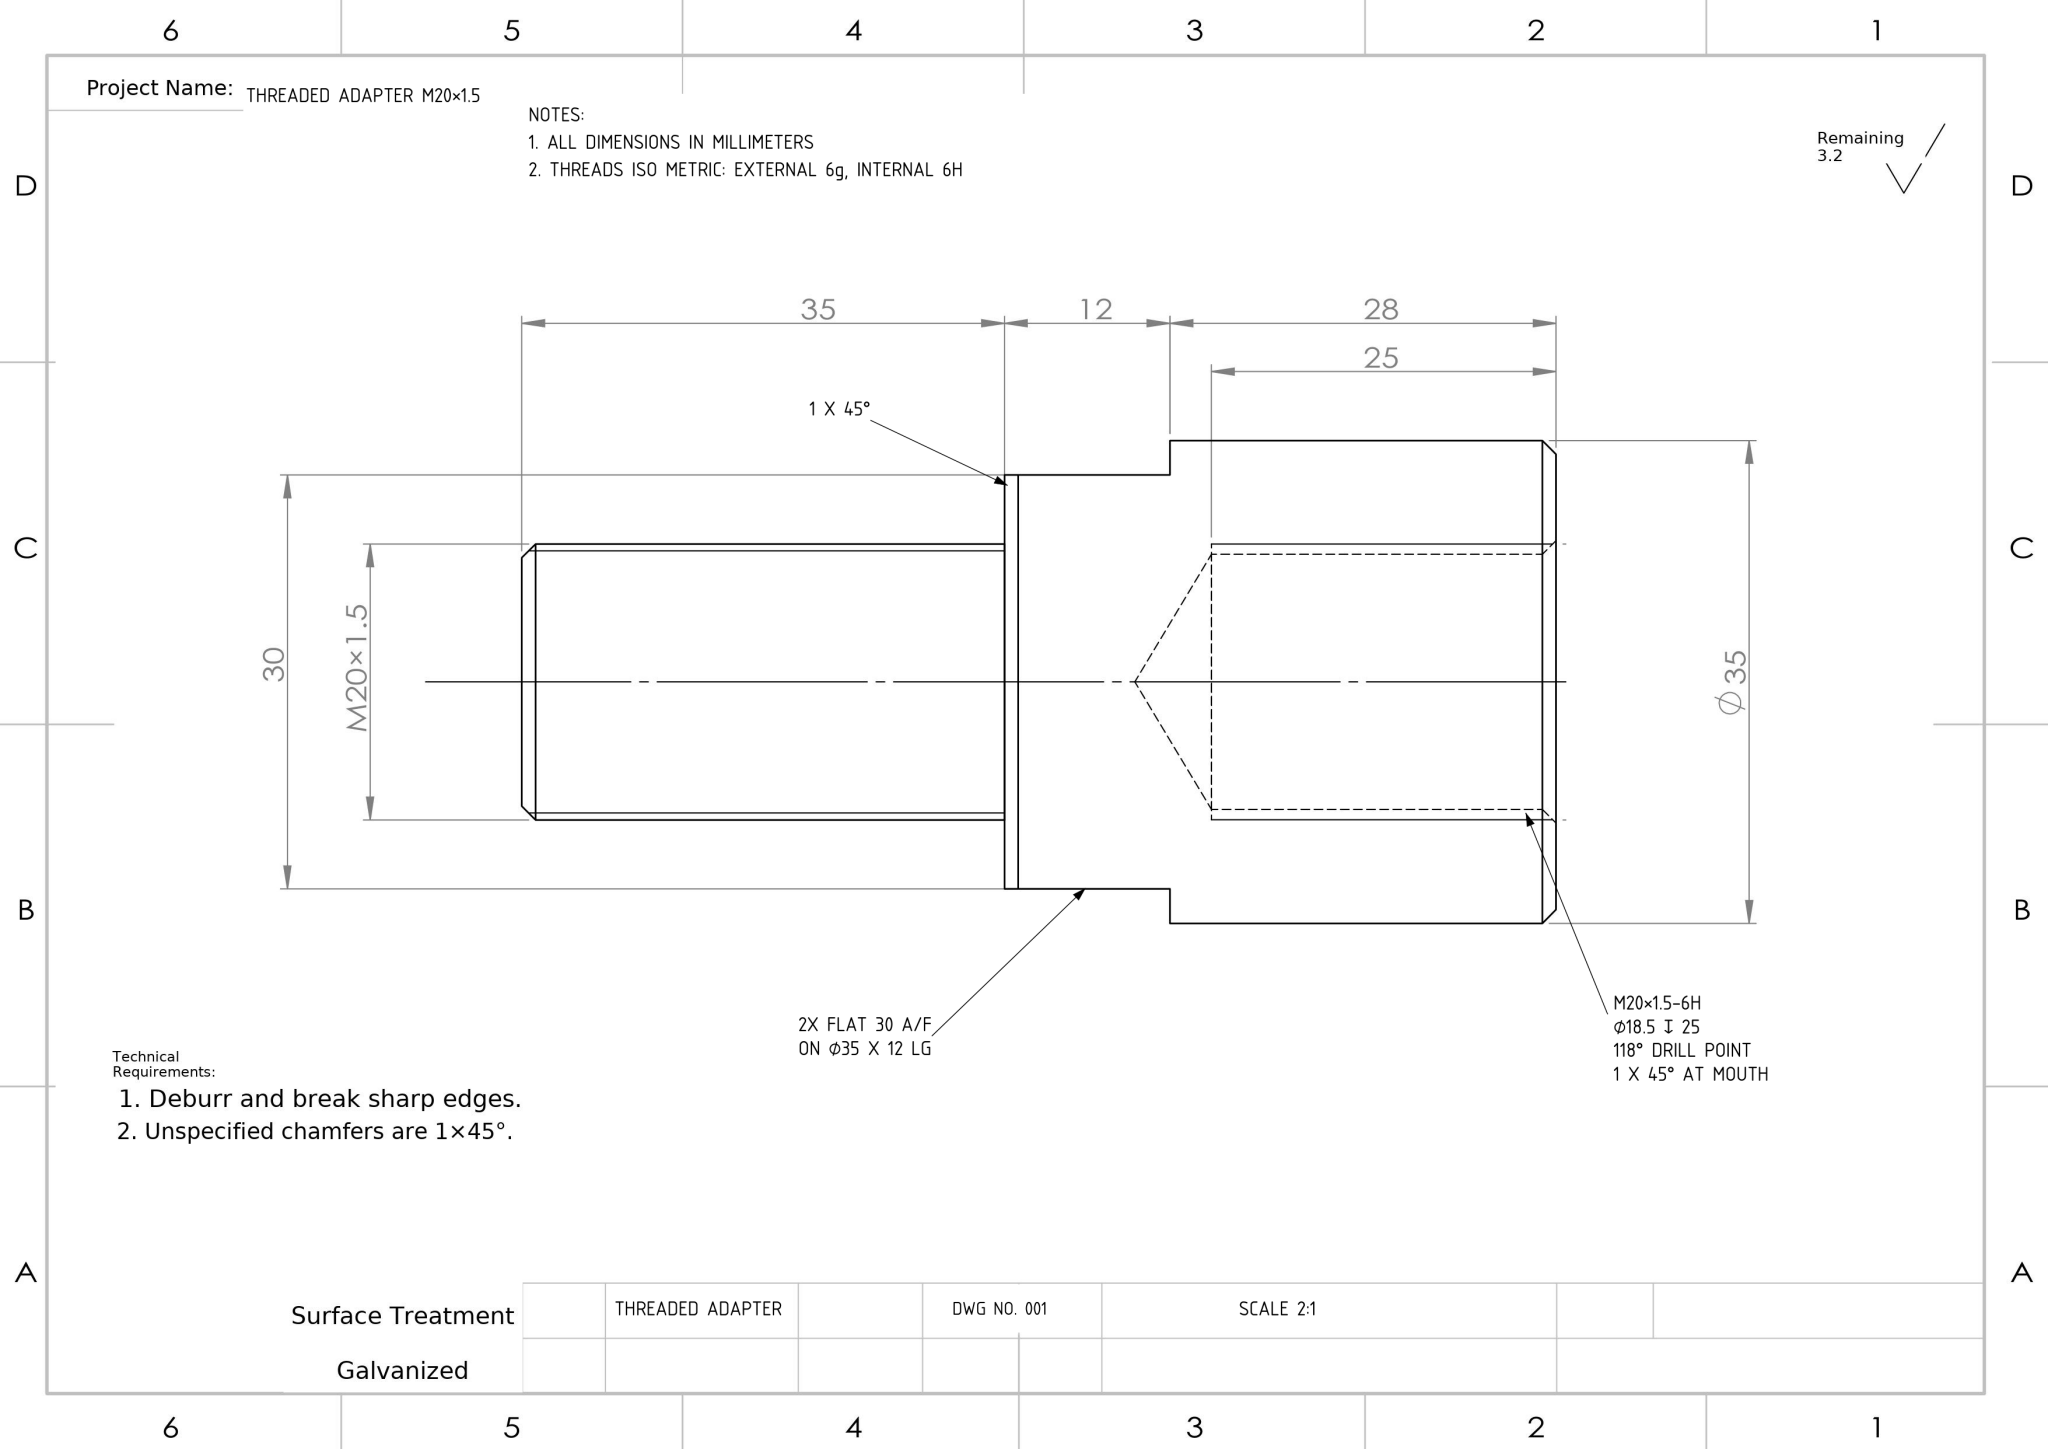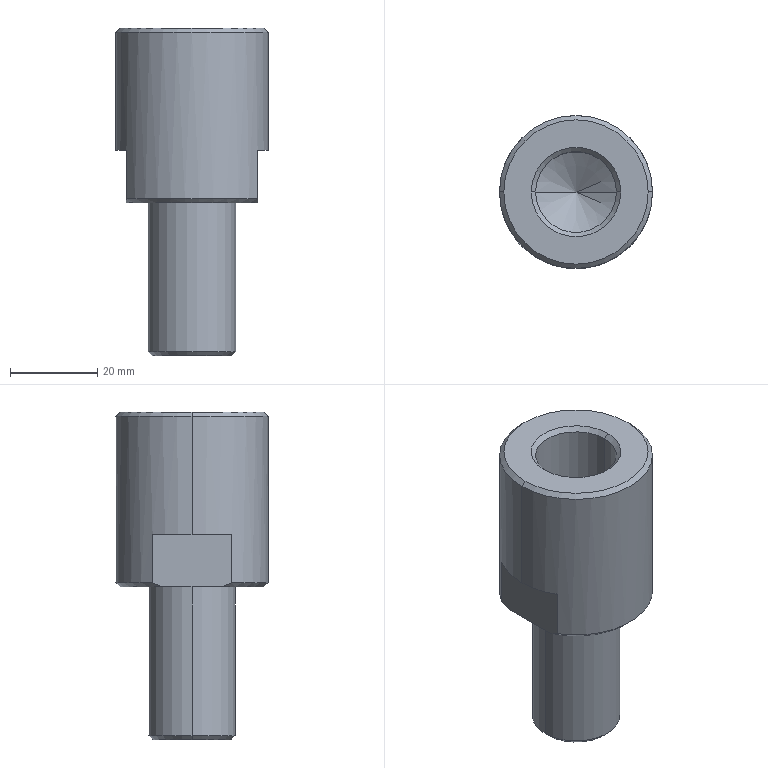Part | NX | mm | 1 solid | 23 faces | box 35 x 35 x 75 mm | volume 41379 mm3 | cone 10 | plane 7 | cylinder 6 | commonest cylinder face diameters 18.5 x2 35 x2 20 x2
STEP:
#1=COLOUR_RGB('',0.7529,0.7529,0.7529);
#2=FILL_AREA_STYLE_COLOUR('',#1);
#3=FILL_AREA_STYLE('',(#2));
#4=SURFACE_STYLE_FILL_AREA(#3);
#5=SURFACE_SIDE_STYLE('',(#4));
#6=SURFACE_STYLE_USAGE(.BOTH.,#5);
#7=PRESENTATION_STYLE_ASSIGNMENT((#6));
#8=CARTESIAN_POINT('',(-9.25,0.,50.));
#9=VERTEX_POINT('',#8);
#10=CARTESIAN_POINT('',(-9.25,0.,74.));
#11=VERTEX_POINT('',#10);
#12=CARTESIAN_POINT('',(-9.25,0.,75.));
#13=DIRECTION('',(0.,0.,1.));
#14=VECTOR('',#13,1000.);
#15=LINE('',#12,#14);
#16=EDGE_CURVE('',#9,#11,#15,.T.);
#17=ORIENTED_EDGE('',*,*,#16,.F.);
#18=CARTESIAN_POINT('',(9.25,0.,50.));
#19=VERTEX_POINT('',#18);
#20=CARTESIAN_POINT('',(0.,0.,50.));
#21=DIRECTION('',(0.,0.,1.));
#22=DIRECTION('',(1.,0.,0.));
#23=AXIS2_PLACEMENT_3D('',#20,#21,#22);
#24=CIRCLE('',#23,9.25);
#25=EDGE_CURVE('',#19,#9,#24,.T.);
#26=ORIENTED_EDGE('',*,*,#25,.F.);
#27=CARTESIAN_POINT('',(9.25,0.,74.));
#28=VERTEX_POINT('',#27);
#29=CARTESIAN_POINT('',(9.25,0.,75.));
#30=DIRECTION('',(0.,0.,1.));
#31=VECTOR('',#30,1000.);
#32=LINE('',#29,#31);
#33=EDGE_CURVE('',#19,#28,#32,.T.);
#34=ORIENTED_EDGE('',*,*,#33,.T.);
#35=CARTESIAN_POINT('',(0.,0.,74.));
#36=DIRECTION('',(0.,0.,1.));
#37=DIRECTION('',(1.,0.,0.));
#38=AXIS2_PLACEMENT_3D('',#35,#36,#37);
#39=CIRCLE('',#38,9.25);
#40=EDGE_CURVE('',#28,#11,#39,.T.);
#41=ORIENTED_EDGE('',*,*,#40,.T.);
#42=EDGE_LOOP('',(#17,#26,#34,#41));
#43=FACE_OUTER_BOUND('',#42,.T.);
#44=CARTESIAN_POINT('',(0.,0.,75.));
#45=DIRECTION('',(0.,0.,1.));
#46=DIRECTION('',(1.,0.,0.));
#47=AXIS2_PLACEMENT_3D('',#44,#45,#46);
#48=CYLINDRICAL_SURFACE('',#47,9.25);
#49=ADVANCED_FACE('',(#43),#48,.F.);
#50=STYLED_ITEM('',(#7),#49);
#51=(LENGTH_UNIT()NAMED_UNIT(*)SI_UNIT(.MILLI.,.METRE.));
#52=UNCERTAINTY_MEASURE_WITH_UNIT(LENGTH_MEASURE(0.00001),#51,'','');
#53=(NAMED_UNIT(*)PLANE_ANGLE_UNIT()SI_UNIT($,.RADIAN.));
#54=(NAMED_UNIT(*)SI_UNIT($,.STERADIAN.)SOLID_ANGLE_UNIT());
#55=(GEOMETRIC_REPRESENTATION_CONTEXT(3)GLOBAL_UNCERTAINTY_ASSIGNED_CONTEXT((#52))GLOBAL_UNIT_ASSIGNED_CONTEXT((#51,#53,#54))REPRESENTATION_CONTEXT('',''));
#56=MECHANICAL_DESIGN_GEOMETRIC_PRESENTATION_REPRESENTATION('',(#50),#55);
#57=PRESENTATION_LAYER_ASSIGNMENT('','',(#50));
#58=COLOUR_RGB('',0.7529,0.7529,0.7529);
#59=FILL_AREA_STYLE_COLOUR('',#58);
#60=FILL_AREA_STYLE('',(#59));
#61=SURFACE_STYLE_FILL_AREA(#60);
#62=SURFACE_SIDE_STYLE('',(#61));
#63=SURFACE_STYLE_USAGE(.BOTH.,#62);
#64=PRESENTATION_STYLE_ASSIGNMENT((#63));
#65=CARTESIAN_POINT('',(0.,0.,50.));
#66=DIRECTION('',(0.,0.,1.));
#67=DIRECTION('',(1.,0.,0.));
#68=AXIS2_PLACEMENT_3D('',#65,#66,#67);
#69=CIRCLE('',#68,9.25);
#70=EDGE_CURVE('',#9,#19,#69,.T.);
#71=ORIENTED_EDGE('',*,*,#70,.F.);
#72=ORIENTED_EDGE('',*,*,#16,.T.);
#73=CARTESIAN_POINT('',(0.,0.,74.));
#74=DIRECTION('',(0.,0.,1.));
#75=DIRECTION('',(1.,0.,0.));
#76=AXIS2_PLACEMENT_3D('',#73,#74,#75);
#77=CIRCLE('',#76,9.25);
#78=EDGE_CURVE('',#11,#28,#77,.T.);
#79=ORIENTED_EDGE('',*,*,#78,.T.);
#80=ORIENTED_EDGE('',*,*,#33,.F.);
#81=EDGE_LOOP('',(#71,#72,#79,#80));
#82=FACE_OUTER_BOUND('',#81,.T.);
#83=CARTESIAN_POINT('',(0.,0.,75.));
#84=DIRECTION('',(0.,0.,1.));
#85=DIRECTION('',(1.,0.,0.));
#86=AXIS2_PLACEMENT_3D('',#83,#84,#85);
#87=CYLINDRICAL_SURFACE('',#86,9.25);
#88=ADVANCED_FACE('',(#82),#87,.F.);
#89=STYLED_ITEM('',(#64),#88);
#90=PRESENTATION_LAYER_ASSIGNMENT('','',(#89));
#91=COLOUR_RGB('',0.7529,0.7529,0.7529);
#92=FILL_AREA_STYLE_COLOUR('',#91);
#93=FILL_AREA_STYLE('',(#92));
#94=SURFACE_STYLE_FILL_AREA(#93);
#95=SURFACE_SIDE_STYLE('',(#94));
#96=SURFACE_STYLE_USAGE(.BOTH.,#95);
#97=PRESENTATION_STYLE_ASSIGNMENT((#96));
#98=ORIENTED_EDGE('',*,*,#78,.F.);
#99=CARTESIAN_POINT('',(-10.25,0.,75.));
#100=VERTEX_POINT('',#99);
#101=CARTESIAN_POINT('',(-9.25,0.,74.));
#102=DIRECTION('',(-0.7071,0.,0.7071));
#103=VECTOR('',#102,1000.);
#104=LINE('',#101,#103);
#105=EDGE_CURVE('',#11,#100,#104,.T.);
#106=ORIENTED_EDGE('',*,*,#105,.T.);
#107=CARTESIAN_POINT('',(10.25,0.,75.));
#108=VERTEX_POINT('',#107);
#109=CARTESIAN_POINT('',(0.,0.,75.));
#110=DIRECTION('',(0.,0.,-1.));
#111=DIRECTION('',(1.,0.,0.));
#112=AXIS2_PLACEMENT_3D('',#109,#110,#111);
#113=CIRCLE('',#112,10.25);
#114=EDGE_CURVE('',#108,#100,#113,.T.);
#115=ORIENTED_EDGE('',*,*,#114,.F.);
#116=CARTESIAN_POINT('',(9.25,0.,74.));
#117=DIRECTION('',(0.7071,0.,0.7071));
#118=VECTOR('',#117,1000.);
#119=LINE('',#116,#118);
#120=EDGE_CURVE('',#28,#108,#119,.T.);
#121=ORIENTED_EDGE('',*,*,#120,.F.);
#122=EDGE_LOOP('',(#98,#106,#115,#121));
#123=FACE_OUTER_BOUND('',#122,.T.);
#124=CARTESIAN_POINT('',(0.,0.,74.));
#125=DIRECTION('',(0.,0.,1.));
#126=DIRECTION('',(1.,0.,0.));
#127=AXIS2_PLACEMENT_3D('',#124,#125,#126);
#128=CONICAL_SURFACE('',#127,9.25,0.7854);
#129=ADVANCED_FACE('',(#123),#128,.F.);
#130=CARTESIAN_POINT('',(-0.,0.,44.442));
#131=VERTEX_POINT('',#130);
#132=CARTESIAN_POINT('',(9.25,0.,50.));
#133=DIRECTION('',(0.8572,0.,0.515));
#134=VECTOR('',#133,1000.);
#135=LINE('',#132,#134);
#136=EDGE_CURVE('',#131,#19,#135,.T.);
#137=ORIENTED_EDGE('',*,*,#136,.F.);
#138=CARTESIAN_POINT('',(-9.25,0.,50.));
#139=DIRECTION('',(-0.8572,0.,0.515));
#140=VECTOR('',#139,1000.);
#141=LINE('',#138,#140);
#142=EDGE_CURVE('',#131,#9,#141,.T.);
#143=ORIENTED_EDGE('',*,*,#142,.T.);
#144=ORIENTED_EDGE('',*,*,#70,.T.);
#145=EDGE_LOOP('',(#137,#143,#144));
#146=FACE_OUTER_BOUND('',#145,.T.);
#147=CARTESIAN_POINT('',(0.,0.,50.));
#148=DIRECTION('',(0.,0.,1.));
#149=DIRECTION('',(1.,0.,0.));
#150=AXIS2_PLACEMENT_3D('',#147,#148,#149);
#151=CONICAL_SURFACE('',#150,9.25,1.03);
#152=ADVANCED_FACE('',(#146),#151,.F.);
#153=CARTESIAN_POINT('',(-9.,0.,0.));
#154=VERTEX_POINT('',#153);
#155=CARTESIAN_POINT('',(9.,0.,0.));
#156=VERTEX_POINT('',#155);
#157=CARTESIAN_POINT('',(0.,0.,0.));
#158=DIRECTION('',(0.,0.,-1.));
#159=DIRECTION('',(1.,0.,0.));
#160=AXIS2_PLACEMENT_3D('',#157,#158,#159);
#161=CIRCLE('',#160,9.);
#162=EDGE_CURVE('',#154,#156,#161,.T.);
#163=ORIENTED_EDGE('',*,*,#162,.F.);
#164=CARTESIAN_POINT('',(-10.,0.,1.));
#165=VERTEX_POINT('',#164);
#166=CARTESIAN_POINT('',(-10.,0.,1.));
#167=DIRECTION('',(-0.7071,0.,0.7071));
#168=VECTOR('',#167,1000.);
#169=LINE('',#166,#168);
#170=EDGE_CURVE('',#154,#165,#169,.T.);
#171=ORIENTED_EDGE('',*,*,#170,.T.);
#172=CARTESIAN_POINT('',(10.,0.,1.));
#173=VERTEX_POINT('',#172);
#174=CARTESIAN_POINT('',(0.,0.,1.));
#175=DIRECTION('',(0.,0.,1.));
#176=DIRECTION('',(1.,0.,0.));
#177=AXIS2_PLACEMENT_3D('',#174,#175,#176);
#178=CIRCLE('',#177,10.);
#179=EDGE_CURVE('',#173,#165,#178,.T.);
#180=ORIENTED_EDGE('',*,*,#179,.F.);
#181=CARTESIAN_POINT('',(10.,0.,1.));
#182=DIRECTION('',(0.7071,0.,0.7071));
#183=VECTOR('',#182,1000.);
#184=LINE('',#181,#183);
#185=EDGE_CURVE('',#156,#173,#184,.T.);
#186=ORIENTED_EDGE('',*,*,#185,.F.);
#187=EDGE_LOOP('',(#163,#171,#180,#186));
#188=FACE_OUTER_BOUND('',#187,.T.);
#189=CARTESIAN_POINT('',(0.,0.,1.));
#190=DIRECTION('',(0.,0.,1.));
#191=DIRECTION('',(1.,0.,0.));
#192=AXIS2_PLACEMENT_3D('',#189,#190,#191);
#193=CONICAL_SURFACE('',#192,10.,0.7854);
#194=ADVANCED_FACE('',(#188),#193,.T.);
#195=CARTESIAN_POINT('',(16.5,0.,75.));
#196=VERTEX_POINT('',#195);
#197=CARTESIAN_POINT('',(-16.5,0.,75.));
#198=VERTEX_POINT('',#197);
#199=CARTESIAN_POINT('',(0.,0.,75.));
#200=DIRECTION('',(0.,0.,1.));
#201=DIRECTION('',(1.,0.,0.));
#202=AXIS2_PLACEMENT_3D('',#199,#200,#201);
#203=CIRCLE('',#202,16.5);
#204=EDGE_CURVE('',#196,#198,#203,.T.);
#205=ORIENTED_EDGE('',*,*,#204,.F.);
#206=CARTESIAN_POINT('',(17.5,0.,74.));
#207=VERTEX_POINT('',#206);
#208=CARTESIAN_POINT('',(16.5,0.,75.));
#209=DIRECTION('',(0.7071,0.,-0.7071));
#210=VECTOR('',#209,1000.);
#211=LINE('',#208,#210);
#212=EDGE_CURVE('',#196,#207,#211,.T.);
#213=ORIENTED_EDGE('',*,*,#212,.T.);
#214=CARTESIAN_POINT('',(-17.5,0.,74.));
#215=VERTEX_POINT('',#214);
#216=CARTESIAN_POINT('',(0.,0.,74.));
#217=DIRECTION('',(0.,0.,-1.));
#218=DIRECTION('',(1.,0.,0.));
#219=AXIS2_PLACEMENT_3D('',#216,#217,#218);
#220=CIRCLE('',#219,17.5);
#221=EDGE_CURVE('',#215,#207,#220,.T.);
#222=ORIENTED_EDGE('',*,*,#221,.F.);
#223=CARTESIAN_POINT('',(-16.5,0.,75.));
#224=DIRECTION('',(-0.7071,0.,-0.7071));
#225=VECTOR('',#224,1000.);
#226=LINE('',#223,#225);
#227=EDGE_CURVE('',#198,#215,#226,.T.);
#228=ORIENTED_EDGE('',*,*,#227,.F.);
#229=EDGE_LOOP('',(#205,#213,#222,#228));
#230=FACE_OUTER_BOUND('',#229,.T.);
#231=CARTESIAN_POINT('',(0.,0.,75.));
#232=DIRECTION('',(0.,0.,-1.));
#233=DIRECTION('',(-1.,0.,0.));
#234=AXIS2_PLACEMENT_3D('',#231,#232,#233);
#235=CONICAL_SURFACE('',#234,16.5,0.7854);
#236=ADVANCED_FACE('',(#230),#235,.T.);
#237=ORIENTED_EDGE('',*,*,#221,.T.);
#238=CARTESIAN_POINT('',(17.5,0.,47.));
#239=VERTEX_POINT('',#238);
#240=CARTESIAN_POINT('',(17.5,0.,75.));
#241=DIRECTION('',(0.,0.,-1.));
#242=VECTOR('',#241,1000.);
#243=LINE('',#240,#242);
#244=EDGE_CURVE('',#207,#239,#243,.T.);
#245=ORIENTED_EDGE('',*,*,#244,.T.);
#246=CARTESIAN_POINT('',(15.,9.014,47.));
#247=VERTEX_POINT('',#246);
#248=CARTESIAN_POINT('',(0.,0.,47.));
#249=DIRECTION('',(0.,0.,1.));
#250=DIRECTION('',(1.,0.,0.));
#251=AXIS2_PLACEMENT_3D('',#248,#249,#250);
#252=CIRCLE('',#251,17.5);
#253=EDGE_CURVE('',#239,#247,#252,.T.);
#254=ORIENTED_EDGE('',*,*,#253,.T.);
#255=CARTESIAN_POINT('',(15.,9.014,36.));
#256=VERTEX_POINT('',#255);
#257=CARTESIAN_POINT('',(15.,9.014,75.));
#258=DIRECTION('',(0.,0.,-1.));
#259=VECTOR('',#258,1000.);
#260=LINE('',#257,#259);
#261=EDGE_CURVE('',#247,#256,#260,.T.);
#262=ORIENTED_EDGE('',*,*,#261,.T.);
#263=CARTESIAN_POINT('',(-15.,9.014,36.));
#264=VERTEX_POINT('',#263);
#265=CARTESIAN_POINT('',(0.,0.,36.));
#266=DIRECTION('',(0.,0.,1.));
#267=DIRECTION('',(1.,0.,0.));
#268=AXIS2_PLACEMENT_3D('',#265,#266,#267);
#269=CIRCLE('',#268,17.5);
#270=EDGE_CURVE('',#256,#264,#269,.T.);
#271=ORIENTED_EDGE('',*,*,#270,.T.);
#272=CARTESIAN_POINT('',(-15.,9.014,47.));
#273=VERTEX_POINT('',#272);
#274=CARTESIAN_POINT('',(-15.,9.014,75.));
#275=DIRECTION('',(0.,0.,1.));
#276=VECTOR('',#275,1000.);
#277=LINE('',#274,#276);
#278=EDGE_CURVE('',#264,#273,#277,.T.);
#279=ORIENTED_EDGE('',*,*,#278,.T.);
#280=CARTESIAN_POINT('',(-17.5,0.,47.));
#281=VERTEX_POINT('',#280);
#282=CARTESIAN_POINT('',(0.,0.,47.));
#283=DIRECTION('',(0.,0.,1.));
#284=DIRECTION('',(1.,0.,0.));
#285=AXIS2_PLACEMENT_3D('',#282,#283,#284);
#286=CIRCLE('',#285,17.5);
#287=EDGE_CURVE('',#273,#281,#286,.T.);
#288=ORIENTED_EDGE('',*,*,#287,.T.);
#289=CARTESIAN_POINT('',(-17.5,0.,75.));
#290=DIRECTION('',(0.,0.,-1.));
#291=VECTOR('',#290,1000.);
#292=LINE('',#289,#291);
#293=EDGE_CURVE('',#215,#281,#292,.T.);
#294=ORIENTED_EDGE('',*,*,#293,.F.);
#295=EDGE_LOOP('',(#237,#245,#254,#262,#271,#279,#288,#294));
#296=FACE_OUTER_BOUND('',#295,.T.);
#297=CARTESIAN_POINT('',(0.,0.,75.));
#298=DIRECTION('',(0.,0.,-1.));
#299=DIRECTION('',(-1.,0.,0.));
#300=AXIS2_PLACEMENT_3D('',#297,#298,#299);
#301=CYLINDRICAL_SURFACE('',#300,17.5);
#302=ADVANCED_FACE('',(#296),#301,.T.);
#303=CARTESIAN_POINT('',(10.,0.,35.));
#304=VERTEX_POINT('',#303);
#305=CARTESIAN_POINT('',(-10.,0.,35.));
#306=VERTEX_POINT('',#305);
#307=CARTESIAN_POINT('',(0.,0.,35.));
#308=DIRECTION('',(0.,0.,1.));
#309=DIRECTION('',(1.,0.,0.));
#310=AXIS2_PLACEMENT_3D('',#307,#308,#309);
#311=CIRCLE('',#310,10.);
#312=EDGE_CURVE('',#304,#306,#311,.T.);
#313=ORIENTED_EDGE('',*,*,#312,.F.);
#314=CARTESIAN_POINT('',(10.,0.,35.));
#315=DIRECTION('',(0.,0.,-1.));
#316=VECTOR('',#315,1000.);
#317=LINE('',#314,#316);
#318=EDGE_CURVE('',#304,#173,#317,.T.);
#319=ORIENTED_EDGE('',*,*,#318,.T.);
#320=ORIENTED_EDGE('',*,*,#179,.T.);
#321=CARTESIAN_POINT('',(-10.,0.,35.));
#322=DIRECTION('',(0.,0.,-1.));
#323=VECTOR('',#322,1000.);
#324=LINE('',#321,#323);
#325=EDGE_CURVE('',#306,#165,#324,.T.);
#326=ORIENTED_EDGE('',*,*,#325,.F.);
#327=EDGE_LOOP('',(#313,#319,#320,#326));
#328=FACE_OUTER_BOUND('',#327,.T.);
#329=CARTESIAN_POINT('',(0.,0.,35.));
#330=DIRECTION('',(0.,0.,-1.));
#331=DIRECTION('',(-1.,0.,0.));
#332=AXIS2_PLACEMENT_3D('',#329,#330,#331);
#333=CYLINDRICAL_SURFACE('',#332,10.);
#334=ADVANCED_FACE('',(#328),#333,.T.);
#335=CARTESIAN_POINT('',(-15.,6.874,35.));
#336=VERTEX_POINT('',#335);
#337=CARTESIAN_POINT('',(-15.,9.014,36.));
#338=CARTESIAN_POINT('',(-15.,8.313,35.639));
#339=CARTESIAN_POINT('',(-15.,7.601,35.303));
#340=CARTESIAN_POINT('',(-15.,6.874,35.));
#341=B_SPLINE_CURVE_WITH_KNOTS('',3,(#337,#338,#339,#340),.UNSPECIFIED.,.F.,.F.,(4,4),(0.03386,0.03623),.UNSPECIFIED.);
#342=EDGE_CURVE('',#264,#336,#341,.T.);
#343=ORIENTED_EDGE('',*,*,#342,.F.);
#344=ORIENTED_EDGE('',*,*,#270,.F.);
#345=CARTESIAN_POINT('',(15.,6.874,35.));
#346=VERTEX_POINT('',#345);
#347=CARTESIAN_POINT('',(15.,6.874,35.));
#348=CARTESIAN_POINT('',(15.,7.604,35.304));
#349=CARTESIAN_POINT('',(15.,8.316,35.64));
#350=CARTESIAN_POINT('',(15.,9.014,36.));
#351=B_SPLINE_CURVE_WITH_KNOTS('',3,(#347,#348,#349,#350),.UNSPECIFIED.,.F.,.F.,(4,4),(0.05039,0.05277),.UNSPECIFIED.);
#352=EDGE_CURVE('',#346,#256,#351,.T.);
#353=ORIENTED_EDGE('',*,*,#352,.F.);
#354=CARTESIAN_POINT('',(0.,0.,35.));
#355=DIRECTION('',(0.,0.,-1.));
#356=DIRECTION('',(1.,0.,0.));
#357=AXIS2_PLACEMENT_3D('',#354,#355,#356);
#358=CIRCLE('',#357,16.5);
#359=EDGE_CURVE('',#336,#346,#358,.T.);
#360=ORIENTED_EDGE('',*,*,#359,.F.);
#361=EDGE_LOOP('',(#343,#344,#353,#360));
#362=FACE_OUTER_BOUND('',#361,.T.);
#363=CARTESIAN_POINT('',(0.,0.,36.));
#364=DIRECTION('',(0.,0.,1.));
#365=DIRECTION('',(1.,0.,0.));
#366=AXIS2_PLACEMENT_3D('',#363,#364,#365);
#367=CONICAL_SURFACE('',#366,17.5,0.7854);
#368=ADVANCED_FACE('',(#362),#367,.T.);
#369=ORIENTED_EDGE('',*,*,#318,.F.);
#370=CARTESIAN_POINT('',(0.,0.,35.));
#371=DIRECTION('',(0.,0.,1.));
#372=DIRECTION('',(1.,0.,0.));
#373=AXIS2_PLACEMENT_3D('',#370,#371,#372);
#374=CIRCLE('',#373,10.);
#375=EDGE_CURVE('',#306,#304,#374,.T.);
#376=ORIENTED_EDGE('',*,*,#375,.F.);
#377=ORIENTED_EDGE('',*,*,#325,.T.);
#378=CARTESIAN_POINT('',(0.,0.,1.));
#379=DIRECTION('',(0.,0.,1.));
#380=DIRECTION('',(1.,0.,0.));
#381=AXIS2_PLACEMENT_3D('',#378,#379,#380);
#382=CIRCLE('',#381,10.);
#383=EDGE_CURVE('',#165,#173,#382,.T.);
#384=ORIENTED_EDGE('',*,*,#383,.T.);
#385=EDGE_LOOP('',(#369,#376,#377,#384));
#386=FACE_OUTER_BOUND('',#385,.T.);
#387=CARTESIAN_POINT('',(0.,0.,35.));
#388=DIRECTION('',(0.,0.,-1.));
#389=DIRECTION('',(-1.,0.,0.));
#390=AXIS2_PLACEMENT_3D('',#387,#388,#389);
#391=CYLINDRICAL_SURFACE('',#390,10.);
#392=ADVANCED_FACE('',(#386),#391,.T.);
#393=CARTESIAN_POINT('',(0.,0.,0.));
#394=DIRECTION('',(0.,0.,-1.));
#395=DIRECTION('',(1.,0.,0.));
#396=AXIS2_PLACEMENT_3D('',#393,#394,#395);
#397=CIRCLE('',#396,9.);
#398=EDGE_CURVE('',#156,#154,#397,.T.);
#399=ORIENTED_EDGE('',*,*,#398,.T.);
#400=ORIENTED_EDGE('',*,*,#162,.T.);
#401=EDGE_LOOP('',(#399,#400));
#402=FACE_OUTER_BOUND('',#401,.T.);
#403=CARTESIAN_POINT('',(0.,0.,0.));
#404=DIRECTION('',(0.,0.,1.));
#405=DIRECTION('',(1.,0.,0.));
#406=AXIS2_PLACEMENT_3D('',#403,#404,#405);
#407=PLANE('',#406);
#408=ADVANCED_FACE('',(#402),#407,.F.);
#409=ORIENTED_EDGE('',*,*,#244,.F.);
#410=CARTESIAN_POINT('',(0.,0.,74.));
#411=DIRECTION('',(0.,0.,-1.));
#412=DIRECTION('',(1.,0.,0.));
#413=AXIS2_PLACEMENT_3D('',#410,#411,#412);
#414=CIRCLE('',#413,17.5);
#415=EDGE_CURVE('',#207,#215,#414,.T.);
#416=ORIENTED_EDGE('',*,*,#415,.T.);
#417=ORIENTED_EDGE('',*,*,#293,.T.);
#418=CARTESIAN_POINT('',(-15.,-9.014,47.));
#419=VERTEX_POINT('',#418);
#420=CARTESIAN_POINT('',(0.,0.,47.));
#421=DIRECTION('',(0.,0.,1.));
#422=DIRECTION('',(1.,0.,0.));
#423=AXIS2_PLACEMENT_3D('',#420,#421,#422);
#424=CIRCLE('',#423,17.5);
#425=EDGE_CURVE('',#281,#419,#424,.T.);
#426=ORIENTED_EDGE('',*,*,#425,.T.);
#427=CARTESIAN_POINT('',(-15.,-9.014,36.));
#428=VERTEX_POINT('',#427);
#429=CARTESIAN_POINT('',(-15.,-9.014,75.));
#430=DIRECTION('',(0.,0.,-1.));
#431=VECTOR('',#430,1000.);
#432=LINE('',#429,#431);
#433=EDGE_CURVE('',#419,#428,#432,.T.);
#434=ORIENTED_EDGE('',*,*,#433,.T.);
#435=CARTESIAN_POINT('',(15.,-9.014,36.));
#436=VERTEX_POINT('',#435);
#437=CARTESIAN_POINT('',(0.,0.,36.));
#438=DIRECTION('',(0.,0.,1.));
#439=DIRECTION('',(1.,0.,0.));
#440=AXIS2_PLACEMENT_3D('',#437,#438,#439);
#441=CIRCLE('',#440,17.5);
#442=EDGE_CURVE('',#428,#436,#441,.T.);
#443=ORIENTED_EDGE('',*,*,#442,.T.);
#444=CARTESIAN_POINT('',(15.,-9.014,47.));
#445=VERTEX_POINT('',#444);
#446=CARTESIAN_POINT('',(15.,-9.014,75.));
#447=DIRECTION('',(0.,0.,1.));
#448=VECTOR('',#447,1000.);
#449=LINE('',#446,#448);
#450=EDGE_CURVE('',#436,#445,#449,.T.);
#451=ORIENTED_EDGE('',*,*,#450,.T.);
#452=CARTESIAN_POINT('',(0.,0.,47.));
#453=DIRECTION('',(0.,0.,1.));
#454=DIRECTION('',(1.,0.,0.));
#455=AXIS2_PLACEMENT_3D('',#452,#453,#454);
#456=CIRCLE('',#455,17.5);
#457=EDGE_CURVE('',#445,#239,#456,.T.);
#458=ORIENTED_EDGE('',*,*,#457,.T.);
#459=EDGE_LOOP('',(#409,#416,#417,#426,#434,#443,#451,#458));
#460=FACE_OUTER_BOUND('',#459,.T.);
#461=CARTESIAN_POINT('',(0.,0.,75.));
#462=DIRECTION('',(0.,0.,-1.));
#463=DIRECTION('',(-1.,0.,0.));
#464=AXIS2_PLACEMENT_3D('',#461,#462,#463);
#465=CYLINDRICAL_SURFACE('',#464,17.5);
#466=ADVANCED_FACE('',(#460),#465,.T.);
#467=ORIENTED_EDGE('',*,*,#114,.T.);
#468=CARTESIAN_POINT('',(0.,0.,75.));
#469=DIRECTION('',(0.,0.,-1.));
#470=DIRECTION('',(1.,0.,0.));
#471=AXIS2_PLACEMENT_3D('',#468,#469,#470);
#472=CIRCLE('',#471,10.25);
#473=EDGE_CURVE('',#100,#108,#472,.T.);
#474=ORIENTED_EDGE('',*,*,#473,.T.);
#475=EDGE_LOOP('',(#467,#474));
#476=FACE_BOUND('',#475,.T.);
#477=CARTESIAN_POINT('',(0.,0.,75.));
#478=DIRECTION('',(0.,0.,1.));
#479=DIRECTION('',(1.,0.,0.));
#480=AXIS2_PLACEMENT_3D('',#477,#478,#479);
#481=CIRCLE('',#480,16.5);
#482=EDGE_CURVE('',#198,#196,#481,.T.);
#483=ORIENTED_EDGE('',*,*,#482,.T.);
#484=ORIENTED_EDGE('',*,*,#204,.T.);
#485=EDGE_LOOP('',(#483,#484));
#486=FACE_OUTER_BOUND('',#485,.T.);
#487=CARTESIAN_POINT('',(0.,0.,75.));
#488=DIRECTION('',(0.,0.,1.));
#489=DIRECTION('',(1.,0.,0.));
#490=AXIS2_PLACEMENT_3D('',#487,#488,#489);
#491=PLANE('',#490);
#492=ADVANCED_FACE('',(#476,#486),#491,.T.);
#493=CARTESIAN_POINT('',(15.,-6.874,35.));
#494=VERTEX_POINT('',#493);
#495=CARTESIAN_POINT('',(-15.,-6.874,35.));
#496=VERTEX_POINT('',#495);
#497=CARTESIAN_POINT('',(0.,0.,35.));
#498=DIRECTION('',(0.,0.,-1.));
#499=DIRECTION('',(1.,0.,0.));
#500=AXIS2_PLACEMENT_3D('',#497,#498,#499);
#501=CIRCLE('',#500,16.5);
#502=EDGE_CURVE('',#494,#496,#501,.T.);
#503=ORIENTED_EDGE('',*,*,#502,.T.);
#504=CARTESIAN_POINT('',(-15.,-17.5,35.));
#505=DIRECTION('',(0.,1.,0.));
#506=VECTOR('',#505,1000.);
#507=LINE('',#504,#506);
#508=EDGE_CURVE('',#496,#336,#507,.T.);
#509=ORIENTED_EDGE('',*,*,#508,.T.);
#510=ORIENTED_EDGE('',*,*,#359,.T.);
#511=CARTESIAN_POINT('',(15.,-17.5,35.));
#512=DIRECTION('',(0.,1.,0.));
#513=VECTOR('',#512,1000.);
#514=LINE('',#511,#513);
#515=EDGE_CURVE('',#494,#346,#514,.T.);
#516=ORIENTED_EDGE('',*,*,#515,.F.);
#517=EDGE_LOOP('',(#503,#509,#510,#516));
#518=FACE_OUTER_BOUND('',#517,.T.);
#519=ORIENTED_EDGE('',*,*,#375,.T.);
#520=ORIENTED_EDGE('',*,*,#312,.T.);
#521=EDGE_LOOP('',(#519,#520));
#522=FACE_BOUND('',#521,.T.);
#523=CARTESIAN_POINT('',(0.,0.,35.));
#524=DIRECTION('',(0.,0.,1.));
#525=DIRECTION('',(1.,0.,0.));
#526=AXIS2_PLACEMENT_3D('',#523,#524,#525);
#527=PLANE('',#526);
#528=ADVANCED_FACE('',(#518,#522),#527,.F.);
#529=ORIENTED_EDGE('',*,*,#212,.F.);
#530=ORIENTED_EDGE('',*,*,#482,.F.);
#531=ORIENTED_EDGE('',*,*,#227,.T.);
#532=ORIENTED_EDGE('',*,*,#415,.F.);
#533=EDGE_LOOP('',(#529,#530,#531,#532));
#534=FACE_OUTER_BOUND('',#533,.T.);
#535=CARTESIAN_POINT('',(0.,0.,75.));
#536=DIRECTION('',(0.,0.,-1.));
#537=DIRECTION('',(-1.,0.,0.));
#538=AXIS2_PLACEMENT_3D('',#535,#536,#537);
#539=CONICAL_SURFACE('',#538,16.5,0.7854);
#540=ADVANCED_FACE('',(#534),#539,.T.);
#541=CARTESIAN_POINT('',(-15.,-6.874,35.));
#542=CARTESIAN_POINT('',(-15.,-7.604,35.304));
#543=CARTESIAN_POINT('',(-15.,-8.316,35.64));
#544=CARTESIAN_POINT('',(-15.,-9.014,36.));
#545=B_SPLINE_CURVE_WITH_KNOTS('',3,(#541,#542,#543,#544),.UNSPECIFIED.,.F.,.F.,(4,4),(0.05039,0.05277),.UNSPECIFIED.);
#546=EDGE_CURVE('',#496,#428,#545,.T.);
#547=ORIENTED_EDGE('',*,*,#546,.F.);
#548=ORIENTED_EDGE('',*,*,#502,.F.);
#549=CARTESIAN_POINT('',(15.,-9.014,36.));
#550=CARTESIAN_POINT('',(15.,-8.313,35.639));
#551=CARTESIAN_POINT('',(15.,-7.601,35.303));
#552=CARTESIAN_POINT('',(15.,-6.874,35.));
#553=B_SPLINE_CURVE_WITH_KNOTS('',3,(#549,#550,#551,#552),.UNSPECIFIED.,.F.,.F.,(4,4),(0.03386,0.03623),.UNSPECIFIED.);
#554=EDGE_CURVE('',#436,#494,#553,.T.);
#555=ORIENTED_EDGE('',*,*,#554,.F.);
#556=ORIENTED_EDGE('',*,*,#442,.F.);
#557=EDGE_LOOP('',(#547,#548,#555,#556));
#558=FACE_OUTER_BOUND('',#557,.T.);
#559=CARTESIAN_POINT('',(0.,0.,36.));
#560=DIRECTION('',(0.,0.,1.));
#561=DIRECTION('',(1.,0.,0.));
#562=AXIS2_PLACEMENT_3D('',#559,#560,#561);
#563=CONICAL_SURFACE('',#562,17.5,0.7854);
#564=ADVANCED_FACE('',(#558),#563,.T.);
#565=ORIENTED_EDGE('',*,*,#170,.F.);
#566=ORIENTED_EDGE('',*,*,#398,.F.);
#567=ORIENTED_EDGE('',*,*,#185,.T.);
#568=ORIENTED_EDGE('',*,*,#383,.F.);
#569=EDGE_LOOP('',(#565,#566,#567,#568));
#570=FACE_OUTER_BOUND('',#569,.T.);
#571=CARTESIAN_POINT('',(0.,0.,1.));
#572=DIRECTION('',(0.,0.,1.));
#573=DIRECTION('',(1.,0.,0.));
#574=AXIS2_PLACEMENT_3D('',#571,#572,#573);
#575=CONICAL_SURFACE('',#574,10.,0.7854);
#576=ADVANCED_FACE('',(#570),#575,.T.);
#577=ORIENTED_EDGE('',*,*,#142,.F.);
#578=ORIENTED_EDGE('',*,*,#136,.T.);
#579=ORIENTED_EDGE('',*,*,#25,.T.);
#580=EDGE_LOOP('',(#577,#578,#579));
#581=FACE_OUTER_BOUND('',#580,.T.);
#582=CARTESIAN_POINT('',(0.,0.,50.));
#583=DIRECTION('',(0.,0.,1.));
#584=DIRECTION('',(1.,0.,0.));
#585=AXIS2_PLACEMENT_3D('',#582,#583,#584);
#586=CONICAL_SURFACE('',#585,9.25,1.03);
#587=ADVANCED_FACE('',(#581),#586,.F.);
#588=ORIENTED_EDGE('',*,*,#105,.F.);
#589=ORIENTED_EDGE('',*,*,#40,.F.);
#590=ORIENTED_EDGE('',*,*,#120,.T.);
#591=ORIENTED_EDGE('',*,*,#473,.F.);
#592=EDGE_LOOP('',(#588,#589,#590,#591));
#593=FACE_OUTER_BOUND('',#592,.T.);
#594=CARTESIAN_POINT('',(0.,0.,74.));
#595=DIRECTION('',(0.,0.,1.));
#596=DIRECTION('',(1.,0.,0.));
#597=AXIS2_PLACEMENT_3D('',#594,#595,#596);
#598=CONICAL_SURFACE('',#597,9.25,0.7854);
#599=ADVANCED_FACE('',(#593),#598,.F.);
#600=CARTESIAN_POINT('',(15.,-17.5,47.));
#601=DIRECTION('',(0.,1.,0.));
#602=VECTOR('',#601,1000.);
#603=LINE('',#600,#602);
#604=EDGE_CURVE('',#445,#247,#603,.T.);
#605=ORIENTED_EDGE('',*,*,#604,.T.);
#606=ORIENTED_EDGE('',*,*,#253,.F.);
#607=ORIENTED_EDGE('',*,*,#457,.F.);
#608=EDGE_LOOP('',(#605,#606,#607));
#609=FACE_OUTER_BOUND('',#608,.T.);
#610=CARTESIAN_POINT('',(38.567,-17.5,47.));
#611=DIRECTION('',(0.,0.,1.));
#612=DIRECTION('',(1.,0.,0.));
#613=AXIS2_PLACEMENT_3D('',#610,#611,#612);
#614=PLANE('',#613);
#615=ADVANCED_FACE('',(#609),#614,.F.);
#616=ORIENTED_EDGE('',*,*,#554,.T.);
#617=ORIENTED_EDGE('',*,*,#515,.T.);
#618=ORIENTED_EDGE('',*,*,#352,.T.);
#619=ORIENTED_EDGE('',*,*,#261,.F.);
#620=ORIENTED_EDGE('',*,*,#604,.F.);
#621=ORIENTED_EDGE('',*,*,#450,.F.);
#622=EDGE_LOOP('',(#616,#617,#618,#619,#620,#621));
#623=FACE_OUTER_BOUND('',#622,.T.);
#624=CARTESIAN_POINT('',(15.,-17.5,47.));
#625=DIRECTION('',(-1.,0.,0.));
#626=DIRECTION('',(0.,0.,1.));
#627=AXIS2_PLACEMENT_3D('',#624,#625,#626);
#628=PLANE('',#627);
#629=ADVANCED_FACE('',(#623),#628,.F.);
#630=CARTESIAN_POINT('',(-15.,-17.5,47.));
#631=DIRECTION('',(0.,1.,0.));
#632=VECTOR('',#631,1000.);
#633=LINE('',#630,#632);
#634=EDGE_CURVE('',#419,#273,#633,.T.);
#635=ORIENTED_EDGE('',*,*,#634,.F.);
#636=ORIENTED_EDGE('',*,*,#425,.F.);
#637=ORIENTED_EDGE('',*,*,#287,.F.);
#638=EDGE_LOOP('',(#635,#636,#637));
#639=FACE_OUTER_BOUND('',#638,.T.);
#640=CARTESIAN_POINT('',(-47.639,-17.5,47.));
#641=DIRECTION('',(0.,0.,1.));
#642=DIRECTION('',(1.,0.,0.));
#643=AXIS2_PLACEMENT_3D('',#640,#641,#642);
#644=PLANE('',#643);
#645=ADVANCED_FACE('',(#639),#644,.F.);
#646=ORIENTED_EDGE('',*,*,#342,.T.);
#647=ORIENTED_EDGE('',*,*,#508,.F.);
#648=ORIENTED_EDGE('',*,*,#546,.T.);
#649=ORIENTED_EDGE('',*,*,#433,.F.);
#650=ORIENTED_EDGE('',*,*,#634,.T.);
#651=ORIENTED_EDGE('',*,*,#278,.F.);
#652=EDGE_LOOP('',(#646,#647,#648,#649,#650,#651));
#653=FACE_OUTER_BOUND('',#652,.T.);
#654=CARTESIAN_POINT('',(-15.,-17.5,47.));
#655=DIRECTION('',(1.,0.,0.));
#656=DIRECTION('',(0.,0.,-1.));
#657=AXIS2_PLACEMENT_3D('',#654,#655,#656);
#658=PLANE('',#657);
#659=ADVANCED_FACE('',(#653),#658,.F.);
#660=CLOSED_SHELL('',(#129,#88,#152,#194,#236,#302,#334,#368,#392,#408,#466,#492,#528,#540,#564,#576,#587,#49,#599,#615,#629,#645,#659));
#661=MANIFOLD_SOLID_BREP('',#660);
#662=CARTESIAN_POINT('',(0.,0.,0.));
#663=DIRECTION('',(0.,0.,1.));
#664=DIRECTION('',(1.,0.,0.));
#665=AXIS2_PLACEMENT_3D('',#662,#663,#664);
#666=(LENGTH_UNIT()NAMED_UNIT(*)SI_UNIT(.MILLI.,.METRE.));
#667=UNCERTAINTY_MEASURE_WITH_UNIT(LENGTH_MEASURE(0.00001),#666,'','');
#668=(NAMED_UNIT(*)PLANE_ANGLE_UNIT()SI_UNIT($,.RADIAN.));
#669=(NAMED_UNIT(*)SI_UNIT($,.STERADIAN.)SOLID_ANGLE_UNIT());
#670=(GEOMETRIC_REPRESENTATION_CONTEXT(3)GLOBAL_UNCERTAINTY_ASSIGNED_CONTEXT((#667))GLOBAL_UNIT_ASSIGNED_CONTEXT((#666,#668,#669))REPRESENTATION_CONTEXT('',''));
#671=ADVANCED_BREP_SHAPE_REPRESENTATION('',(#661,#665),#670);
#672=STYLED_ITEM('',(#97),#671);
#673=(LENGTH_UNIT()NAMED_UNIT(*)SI_UNIT(.MILLI.,.METRE.));
#674=UNCERTAINTY_MEASURE_WITH_UNIT(LENGTH_MEASURE(0.00001),#673,'','');
#675=(NAMED_UNIT(*)PLANE_ANGLE_UNIT()SI_UNIT($,.RADIAN.));
#676=(NAMED_UNIT(*)SI_UNIT($,.STERADIAN.)SOLID_ANGLE_UNIT());
#677=(GEOMETRIC_REPRESENTATION_CONTEXT(3)GLOBAL_UNCERTAINTY_ASSIGNED_CONTEXT((#674))GLOBAL_UNIT_ASSIGNED_CONTEXT((#673,#675,#676))REPRESENTATION_CONTEXT('',''));
#678=MECHANICAL_DESIGN_GEOMETRIC_PRESENTATION_REPRESENTATION('',(#672),#677);
#679=PRESENTATION_LAYER_ASSIGNMENT('','',(#672));
#680=COLOUR_RGB('',0.7765,0.7765,0.8196);
#681=FILL_AREA_STYLE_COLOUR('',#680);
#682=FILL_AREA_STYLE('',(#681));
#683=SURFACE_STYLE_FILL_AREA(#682);
#684=SURFACE_SIDE_STYLE('',(#683));
#685=SURFACE_STYLE_USAGE(.BOTH.,#684);
#686=PRESENTATION_STYLE_ASSIGNMENT((#685));
#687=STYLED_ITEM('',(#686),#334);
#688=(LENGTH_UNIT()NAMED_UNIT(*)SI_UNIT(.MILLI.,.METRE.));
#689=UNCERTAINTY_MEASURE_WITH_UNIT(LENGTH_MEASURE(0.00001),#688,'','');
#690=(NAMED_UNIT(*)PLANE_ANGLE_UNIT()SI_UNIT($,.RADIAN.));
#691=(NAMED_UNIT(*)SI_UNIT($,.STERADIAN.)SOLID_ANGLE_UNIT());
#692=(GEOMETRIC_REPRESENTATION_CONTEXT(3)GLOBAL_UNCERTAINTY_ASSIGNED_CONTEXT((#689))GLOBAL_UNIT_ASSIGNED_CONTEXT((#688,#690,#691))REPRESENTATION_CONTEXT('',''));
#693=MECHANICAL_DESIGN_GEOMETRIC_PRESENTATION_REPRESENTATION('',(#687),#692);
#694=PRESENTATION_LAYER_ASSIGNMENT('','',(#687));
#695=COLOUR_RGB('',0.7529,0.7529,0.7529);
#696=FILL_AREA_STYLE_COLOUR('',#695);
#697=FILL_AREA_STYLE('',(#696));
#698=SURFACE_STYLE_FILL_AREA(#697);
#699=SURFACE_SIDE_STYLE('',(#698));
#700=SURFACE_STYLE_USAGE(.BOTH.,#699);
#701=PRESENTATION_STYLE_ASSIGNMENT((#700));
#702=STYLED_ITEM('',(#701),#661);
#703=PRESENTATION_LAYER_ASSIGNMENT('','',(#702));
#704=(LENGTH_UNIT()NAMED_UNIT(*)SI_UNIT(.MILLI.,.METRE.));
#705=UNCERTAINTY_MEASURE_WITH_UNIT(LENGTH_MEASURE(0.00001),#704,'','');
#706=(NAMED_UNIT(*)PLANE_ANGLE_UNIT()SI_UNIT($,.RADIAN.));
#707=(NAMED_UNIT(*)SI_UNIT($,.STERADIAN.)SOLID_ANGLE_UNIT());
#708=(GEOMETRIC_REPRESENTATION_CONTEXT(3)GLOBAL_UNCERTAINTY_ASSIGNED_CONTEXT((#705))GLOBAL_UNIT_ASSIGNED_CONTEXT((#704,#706,#707))REPRESENTATION_CONTEXT('',''));
#709=MECHANICAL_DESIGN_GEOMETRIC_PRESENTATION_REPRESENTATION('',(#702),#708);
#710=(LENGTH_UNIT()NAMED_UNIT(*)SI_UNIT(.MILLI.,.METRE.));
#711=UNCERTAINTY_MEASURE_WITH_UNIT(LENGTH_MEASURE(0.00001),#710,'','');
#712=(NAMED_UNIT(*)PLANE_ANGLE_UNIT()SI_UNIT($,.RADIAN.));
#713=(NAMED_UNIT(*)SI_UNIT($,.STERADIAN.)SOLID_ANGLE_UNIT());
#714=(GEOMETRIC_REPRESENTATION_CONTEXT(3)GLOBAL_UNCERTAINTY_ASSIGNED_CONTEXT((#711))GLOBAL_UNIT_ASSIGNED_CONTEXT((#710,#712,#713))REPRESENTATION_CONTEXT('',''));
#715=MECHANICAL_DESIGN_GEOMETRIC_PRESENTATION_REPRESENTATION('',(#89),#714);
#716=COLOUR_RGB('',0.7765,0.7765,0.8196);
#717=FILL_AREA_STYLE_COLOUR('',#716);
#718=FILL_AREA_STYLE('',(#717));
#719=SURFACE_STYLE_FILL_AREA(#718);
#720=SURFACE_SIDE_STYLE('',(#719));
#721=SURFACE_STYLE_USAGE(.BOTH.,#720);
#722=PRESENTATION_STYLE_ASSIGNMENT((#721));
#723=STYLED_ITEM('',(#722),#392);
#724=PRESENTATION_LAYER_ASSIGNMENT('','',(#723));
#725=(LENGTH_UNIT()NAMED_UNIT(*)SI_UNIT(.MILLI.,.METRE.));
#726=UNCERTAINTY_MEASURE_WITH_UNIT(LENGTH_MEASURE(0.00001),#725,'','');
#727=(NAMED_UNIT(*)PLANE_ANGLE_UNIT()SI_UNIT($,.RADIAN.));
#728=(NAMED_UNIT(*)SI_UNIT($,.STERADIAN.)SOLID_ANGLE_UNIT());
#729=(GEOMETRIC_REPRESENTATION_CONTEXT(3)GLOBAL_UNCERTAINTY_ASSIGNED_CONTEXT((#726))GLOBAL_UNIT_ASSIGNED_CONTEXT((#725,#727,#728))REPRESENTATION_CONTEXT('',''));
#730=MECHANICAL_DESIGN_GEOMETRIC_PRESENTATION_REPRESENTATION('',(#723),#729);